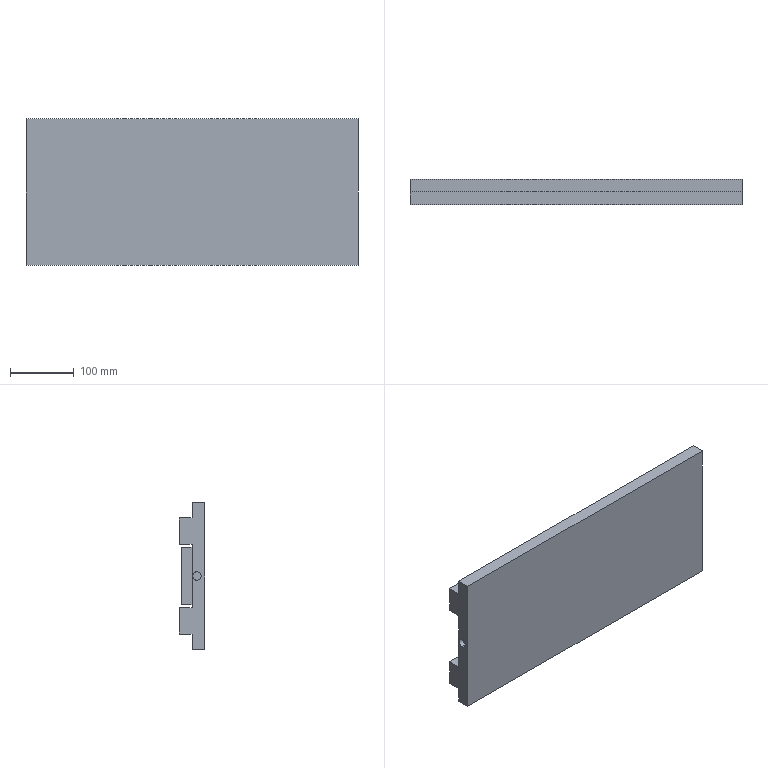Component | SolidWorks | X-AxisSupportBase-1 | 1 solid | 40 faces | box 520 x 40 x 230 mm | volume 3293748 mm3 | plane 27 | cylinder 13 | commonest cylinder face diameters 5.084 x8 13.093 x2 2.946 x2 49.4 x1
STEP:
#1=COLOUR_RGB('',0.7922,0.8196,0.9333);
#2=FILL_AREA_STYLE_COLOUR('',#1);
#3=FILL_AREA_STYLE('',(#2));
#4=SURFACE_STYLE_FILL_AREA(#3);
#5=SURFACE_SIDE_STYLE('',(#4));
#6=SURFACE_STYLE_USAGE(.BOTH.,#5);
#7=PRESENTATION_STYLE_ASSIGNMENT((#6));
#8=CARTESIAN_POINT('',(6.767,1.417,1.368));
#9=VERTEX_POINT('',#8);
#10=CARTESIAN_POINT('',(6.767,1.417,1.568));
#11=VERTEX_POINT('',#10);
#12=CARTESIAN_POINT('',(6.767,1.417,1.468));
#13=DIRECTION('',(0.,1.,0.));
#14=DIRECTION('',(0.,0.,1.));
#15=AXIS2_PLACEMENT_3D('',#12,#13,#14);
#16=CIRCLE('',#15,0.1001);
#17=EDGE_CURVE('',#9,#11,#16,.T.);
#18=ORIENTED_EDGE('',*,*,#17,.T.);
#19=CARTESIAN_POINT('',(6.767,0.7874,1.568));
#20=VERTEX_POINT('',#19);
#21=CARTESIAN_POINT('',(6.767,1.417,1.568));
#22=DIRECTION('',(0.,-1.,0.));
#23=VECTOR('',#22,39.37);
#24=LINE('',#21,#23);
#25=EDGE_CURVE('',#11,#20,#24,.T.);
#26=ORIENTED_EDGE('',*,*,#25,.T.);
#27=CARTESIAN_POINT('',(6.767,0.7874,1.368));
#28=VERTEX_POINT('',#27);
#29=CARTESIAN_POINT('',(6.767,0.7874,1.468));
#30=DIRECTION('',(0.,1.,0.));
#31=DIRECTION('',(0.,0.,1.));
#32=AXIS2_PLACEMENT_3D('',#29,#30,#31);
#33=CIRCLE('',#32,0.1001);
#34=EDGE_CURVE('',#28,#20,#33,.T.);
#35=ORIENTED_EDGE('',*,*,#34,.F.);
#36=CARTESIAN_POINT('',(6.767,1.417,1.368));
#37=DIRECTION('',(0.,-1.,0.));
#38=VECTOR('',#37,39.37);
#39=LINE('',#36,#38);
#40=EDGE_CURVE('',#9,#28,#39,.T.);
#41=ORIENTED_EDGE('',*,*,#40,.F.);
#42=EDGE_LOOP('',(#18,#26,#35,#41));
#43=FACE_OUTER_BOUND('',#42,.T.);
#44=CARTESIAN_POINT('',(6.767,1.417,1.468));
#45=DIRECTION('',(0.,-1.,0.));
#46=DIRECTION('',(0.,0.,-1.));
#47=AXIS2_PLACEMENT_3D('',#44,#45,#46);
#48=CYLINDRICAL_SURFACE('',#47,0.1001);
#49=ADVANCED_FACE('',(#43),#48,.F.);
#50=CARTESIAN_POINT('',(6.208,1.417,1.368));
#51=VERTEX_POINT('',#50);
#52=CARTESIAN_POINT('',(6.208,1.417,1.568));
#53=VERTEX_POINT('',#52);
#54=CARTESIAN_POINT('',(6.208,1.417,1.468));
#55=DIRECTION('',(0.,1.,0.));
#56=DIRECTION('',(0.,0.,1.));
#57=AXIS2_PLACEMENT_3D('',#54,#55,#56);
#58=CIRCLE('',#57,0.1001);
#59=EDGE_CURVE('',#51,#53,#58,.T.);
#60=ORIENTED_EDGE('',*,*,#59,.T.);
#61=CARTESIAN_POINT('',(6.208,0.7874,1.568));
#62=VERTEX_POINT('',#61);
#63=CARTESIAN_POINT('',(6.208,1.417,1.568));
#64=DIRECTION('',(0.,-1.,0.));
#65=VECTOR('',#64,39.37);
#66=LINE('',#63,#65);
#67=EDGE_CURVE('',#53,#62,#66,.T.);
#68=ORIENTED_EDGE('',*,*,#67,.T.);
#69=CARTESIAN_POINT('',(6.208,0.7874,1.368));
#70=VERTEX_POINT('',#69);
#71=CARTESIAN_POINT('',(6.208,0.7874,1.468));
#72=DIRECTION('',(0.,1.,0.));
#73=DIRECTION('',(0.,0.,1.));
#74=AXIS2_PLACEMENT_3D('',#71,#72,#73);
#75=CIRCLE('',#74,0.1001);
#76=EDGE_CURVE('',#70,#62,#75,.T.);
#77=ORIENTED_EDGE('',*,*,#76,.F.);
#78=CARTESIAN_POINT('',(6.208,1.417,1.368));
#79=DIRECTION('',(0.,-1.,0.));
#80=VECTOR('',#79,39.37);
#81=LINE('',#78,#80);
#82=EDGE_CURVE('',#51,#70,#81,.T.);
#83=ORIENTED_EDGE('',*,*,#82,.F.);
#84=EDGE_LOOP('',(#60,#68,#77,#83));
#85=FACE_OUTER_BOUND('',#84,.T.);
#86=CARTESIAN_POINT('',(6.208,1.417,1.468));
#87=DIRECTION('',(0.,-1.,0.));
#88=DIRECTION('',(0.,0.,-1.));
#89=AXIS2_PLACEMENT_3D('',#86,#87,#88);
#90=CYLINDRICAL_SURFACE('',#89,0.1001);
#91=ADVANCED_FACE('',(#85),#90,.F.);
#92=CARTESIAN_POINT('',(6.767,1.417,-1.568));
#93=VERTEX_POINT('',#92);
#94=CARTESIAN_POINT('',(6.767,1.417,-1.368));
#95=VERTEX_POINT('',#94);
#96=CARTESIAN_POINT('',(6.767,1.417,-1.468));
#97=DIRECTION('',(0.,1.,0.));
#98=DIRECTION('',(0.,0.,1.));
#99=AXIS2_PLACEMENT_3D('',#96,#97,#98);
#100=CIRCLE('',#99,0.1001);
#101=EDGE_CURVE('',#93,#95,#100,.T.);
#102=ORIENTED_EDGE('',*,*,#101,.T.);
#103=CARTESIAN_POINT('',(6.767,0.7874,-1.368));
#104=VERTEX_POINT('',#103);
#105=CARTESIAN_POINT('',(6.767,1.417,-1.368));
#106=DIRECTION('',(0.,-1.,0.));
#107=VECTOR('',#106,39.37);
#108=LINE('',#105,#107);
#109=EDGE_CURVE('',#95,#104,#108,.T.);
#110=ORIENTED_EDGE('',*,*,#109,.T.);
#111=CARTESIAN_POINT('',(6.767,0.7874,-1.568));
#112=VERTEX_POINT('',#111);
#113=CARTESIAN_POINT('',(6.767,0.7874,-1.468));
#114=DIRECTION('',(0.,1.,0.));
#115=DIRECTION('',(0.,0.,1.));
#116=AXIS2_PLACEMENT_3D('',#113,#114,#115);
#117=CIRCLE('',#116,0.1001);
#118=EDGE_CURVE('',#112,#104,#117,.T.);
#119=ORIENTED_EDGE('',*,*,#118,.F.);
#120=CARTESIAN_POINT('',(6.767,1.417,-1.568));
#121=DIRECTION('',(0.,-1.,0.));
#122=VECTOR('',#121,39.37);
#123=LINE('',#120,#122);
#124=EDGE_CURVE('',#93,#112,#123,.T.);
#125=ORIENTED_EDGE('',*,*,#124,.F.);
#126=EDGE_LOOP('',(#102,#110,#119,#125));
#127=FACE_OUTER_BOUND('',#126,.T.);
#128=CARTESIAN_POINT('',(6.767,1.417,-1.468));
#129=DIRECTION('',(0.,-1.,0.));
#130=DIRECTION('',(0.,0.,-1.));
#131=AXIS2_PLACEMENT_3D('',#128,#129,#130);
#132=CYLINDRICAL_SURFACE('',#131,0.1001);
#133=ADVANCED_FACE('',(#127),#132,.F.);
#134=CARTESIAN_POINT('',(6.208,1.417,-1.568));
#135=VERTEX_POINT('',#134);
#136=CARTESIAN_POINT('',(6.208,1.417,-1.368));
#137=VERTEX_POINT('',#136);
#138=CARTESIAN_POINT('',(6.208,1.417,-1.468));
#139=DIRECTION('',(0.,1.,0.));
#140=DIRECTION('',(0.,0.,1.));
#141=AXIS2_PLACEMENT_3D('',#138,#139,#140);
#142=CIRCLE('',#141,0.1001);
#143=EDGE_CURVE('',#135,#137,#142,.T.);
#144=ORIENTED_EDGE('',*,*,#143,.T.);
#145=CARTESIAN_POINT('',(6.208,0.7874,-1.368));
#146=VERTEX_POINT('',#145);
#147=CARTESIAN_POINT('',(6.208,1.417,-1.368));
#148=DIRECTION('',(0.,-1.,0.));
#149=VECTOR('',#148,39.37);
#150=LINE('',#147,#149);
#151=EDGE_CURVE('',#137,#146,#150,.T.);
#152=ORIENTED_EDGE('',*,*,#151,.T.);
#153=CARTESIAN_POINT('',(6.208,0.7874,-1.568));
#154=VERTEX_POINT('',#153);
#155=CARTESIAN_POINT('',(6.208,0.7874,-1.468));
#156=DIRECTION('',(0.,1.,0.));
#157=DIRECTION('',(0.,0.,1.));
#158=AXIS2_PLACEMENT_3D('',#155,#156,#157);
#159=CIRCLE('',#158,0.1001);
#160=EDGE_CURVE('',#154,#146,#159,.T.);
#161=ORIENTED_EDGE('',*,*,#160,.F.);
#162=CARTESIAN_POINT('',(6.208,1.417,-1.568));
#163=DIRECTION('',(0.,-1.,0.));
#164=VECTOR('',#163,39.37);
#165=LINE('',#162,#164);
#166=EDGE_CURVE('',#135,#154,#165,.T.);
#167=ORIENTED_EDGE('',*,*,#166,.F.);
#168=EDGE_LOOP('',(#144,#152,#161,#167));
#169=FACE_OUTER_BOUND('',#168,.T.);
#170=CARTESIAN_POINT('',(6.208,1.417,-1.468));
#171=DIRECTION('',(0.,-1.,0.));
#172=DIRECTION('',(0.,0.,-1.));
#173=AXIS2_PLACEMENT_3D('',#170,#171,#172);
#174=CYLINDRICAL_SURFACE('',#173,0.1001);
#175=ADVANCED_FACE('',(#169),#174,.F.);
#176=CARTESIAN_POINT('',(-10.591,0.4812,-0.2577));
#177=VERTEX_POINT('',#176);
#178=CARTESIAN_POINT('',(-10.591,0.4812,0.2577));
#179=VERTEX_POINT('',#178);
#180=CARTESIAN_POINT('',(-10.591,0.4812,0.));
#181=DIRECTION('',(-1.,0.,0.));
#182=DIRECTION('',(0.,0.,1.));
#183=AXIS2_PLACEMENT_3D('',#180,#181,#182);
#184=CIRCLE('',#183,0.2577);
#185=EDGE_CURVE('',#177,#179,#184,.T.);
#186=ORIENTED_EDGE('',*,*,#185,.F.);
#187=CARTESIAN_POINT('',(-10.906,0.4812,-0.2577));
#188=VERTEX_POINT('',#187);
#189=CARTESIAN_POINT('',(-10.591,0.4812,-0.2577));
#190=DIRECTION('',(-1.,0.,0.));
#191=VECTOR('',#190,39.37);
#192=LINE('',#189,#191);
#193=EDGE_CURVE('',#177,#188,#192,.T.);
#194=ORIENTED_EDGE('',*,*,#193,.T.);
#195=CARTESIAN_POINT('',(-10.906,0.4812,0.2577));
#196=VERTEX_POINT('',#195);
#197=CARTESIAN_POINT('',(-10.906,0.4812,0.));
#198=DIRECTION('',(-1.,0.,0.));
#199=DIRECTION('',(0.,0.,1.));
#200=AXIS2_PLACEMENT_3D('',#197,#198,#199);
#201=CIRCLE('',#200,0.2577);
#202=EDGE_CURVE('',#188,#196,#201,.T.);
#203=ORIENTED_EDGE('',*,*,#202,.T.);
#204=CARTESIAN_POINT('',(-10.591,0.4812,0.2577));
#205=DIRECTION('',(-1.,0.,0.));
#206=VECTOR('',#205,39.37);
#207=LINE('',#204,#206);
#208=EDGE_CURVE('',#179,#196,#207,.T.);
#209=ORIENTED_EDGE('',*,*,#208,.F.);
#210=EDGE_LOOP('',(#186,#194,#203,#209));
#211=FACE_OUTER_BOUND('',#210,.T.);
#212=CARTESIAN_POINT('',(-10.591,0.4812,0.));
#213=DIRECTION('',(-1.,0.,0.));
#214=DIRECTION('',(0.,0.,1.));
#215=AXIS2_PLACEMENT_3D('',#212,#213,#214);
#216=CYLINDRICAL_SURFACE('',#215,0.2577);
#217=ADVANCED_FACE('',(#211),#216,.F.);
#218=CARTESIAN_POINT('',(7.039,1.417,0.191));
#219=VERTEX_POINT('',#218);
#220=CARTESIAN_POINT('',(7.039,1.417,-0.191));
#221=VERTEX_POINT('',#220);
#222=CARTESIAN_POINT('',(7.039,2.371,0.));
#223=DIRECTION('',(1.,0.,0.));
#224=DIRECTION('',(0.,0.,-1.));
#225=AXIS2_PLACEMENT_3D('',#222,#223,#224);
#226=CIRCLE('',#225,0.9724);
#227=EDGE_CURVE('',#219,#221,#226,.T.);
#228=ORIENTED_EDGE('',*,*,#227,.F.);
#229=CARTESIAN_POINT('',(7.039,1.417,1.781));
#230=VERTEX_POINT('',#229);
#231=CARTESIAN_POINT('',(7.039,1.417,-1.083));
#232=DIRECTION('',(0.,0.,-1.));
#233=VECTOR('',#232,39.37);
#234=LINE('',#231,#233);
#235=EDGE_CURVE('',#230,#219,#234,.T.);
#236=ORIENTED_EDGE('',*,*,#235,.F.);
#237=CARTESIAN_POINT('',(7.039,0.7874,1.781));
#238=VERTEX_POINT('',#237);
#239=CARTESIAN_POINT('',(7.039,1.417,1.781));
#240=DIRECTION('',(0.,-1.,0.));
#241=VECTOR('',#240,39.37);
#242=LINE('',#239,#241);
#243=EDGE_CURVE('',#230,#238,#242,.T.);
#244=ORIENTED_EDGE('',*,*,#243,.T.);
#245=CARTESIAN_POINT('',(7.039,0.7874,-1.781));
#246=VERTEX_POINT('',#245);
#247=CARTESIAN_POINT('',(7.039,0.7874,1.791));
#248=DIRECTION('',(0.,0.,-1.));
#249=VECTOR('',#248,39.37);
#250=LINE('',#247,#249);
#251=EDGE_CURVE('',#238,#246,#250,.T.);
#252=ORIENTED_EDGE('',*,*,#251,.T.);
#253=CARTESIAN_POINT('',(7.039,1.417,-1.781));
#254=VERTEX_POINT('',#253);
#255=CARTESIAN_POINT('',(7.039,1.417,-1.781));
#256=DIRECTION('',(0.,1.,0.));
#257=VECTOR('',#256,39.37);
#258=LINE('',#255,#257);
#259=EDGE_CURVE('',#246,#254,#258,.T.);
#260=ORIENTED_EDGE('',*,*,#259,.T.);
#261=CARTESIAN_POINT('',(7.039,1.417,-1.083));
#262=DIRECTION('',(0.,0.,-1.));
#263=VECTOR('',#262,39.37);
#264=LINE('',#261,#263);
#265=EDGE_CURVE('',#221,#254,#264,.T.);
#266=ORIENTED_EDGE('',*,*,#265,.F.);
#267=EDGE_LOOP('',(#228,#236,#244,#252,#260,#266));
#268=FACE_OUTER_BOUND('',#267,.T.);
#269=CARTESIAN_POINT('',(7.039,1.417,1.791));
#270=DIRECTION('',(-1.,0.,0.));
#271=DIRECTION('',(0.,0.,1.));
#272=AXIS2_PLACEMENT_3D('',#269,#270,#271);
#273=PLANE('',#272);
#274=ADVANCED_FACE('',(#268),#273,.F.);
#275=CARTESIAN_POINT('',(-10.906,0.7874,4.528));
#276=VERTEX_POINT('',#275);
#277=CARTESIAN_POINT('',(9.567,0.7874,4.528));
#278=VERTEX_POINT('',#277);
#279=CARTESIAN_POINT('',(0.,0.7874,4.528));
#280=DIRECTION('',(1.,0.,0.));
#281=VECTOR('',#280,39.37);
#282=LINE('',#279,#281);
#283=EDGE_CURVE('',#276,#278,#282,.T.);
#284=ORIENTED_EDGE('',*,*,#283,.T.);
#285=CARTESIAN_POINT('',(9.567,0.7874,3.579));
#286=VERTEX_POINT('',#285);
#287=CARTESIAN_POINT('',(9.567,0.7874,0.));
#288=DIRECTION('',(0.,0.,1.));
#289=VECTOR('',#288,39.37);
#290=LINE('',#287,#289);
#291=EDGE_CURVE('',#286,#278,#290,.T.);
#292=ORIENTED_EDGE('',*,*,#291,.F.);
#293=CARTESIAN_POINT('',(-10.906,0.7874,3.579));
#294=VERTEX_POINT('',#293);
#295=CARTESIAN_POINT('',(0.,0.7874,3.579));
#296=DIRECTION('',(1.,0.,0.));
#297=VECTOR('',#296,39.37);
#298=LINE('',#295,#297);
#299=EDGE_CURVE('',#294,#286,#298,.T.);
#300=ORIENTED_EDGE('',*,*,#299,.F.);
#301=CARTESIAN_POINT('',(-10.906,0.7874,4.528));
#302=DIRECTION('',(0.,0.,1.));
#303=VECTOR('',#302,39.37);
#304=LINE('',#301,#303);
#305=EDGE_CURVE('',#294,#276,#304,.T.);
#306=ORIENTED_EDGE('',*,*,#305,.T.);
#307=EDGE_LOOP('',(#284,#292,#300,#306));
#308=FACE_OUTER_BOUND('',#307,.T.);
#309=CARTESIAN_POINT('',(0.,0.7874,0.));
#310=DIRECTION('',(0.,-1.,0.));
#311=DIRECTION('',(0.,0.,-1.));
#312=AXIS2_PLACEMENT_3D('',#309,#310,#311);
#313=PLANE('',#312);
#314=ADVANCED_FACE('',(#308),#313,.F.);
#315=CARTESIAN_POINT('',(9.567,0.7874,-4.528));
#316=VERTEX_POINT('',#315);
#317=CARTESIAN_POINT('',(-10.906,0.7874,-4.528));
#318=VERTEX_POINT('',#317);
#319=CARTESIAN_POINT('',(-0.,0.7874,-4.528));
#320=DIRECTION('',(-1.,0.,0.));
#321=VECTOR('',#320,39.37);
#322=LINE('',#319,#321);
#323=EDGE_CURVE('',#316,#318,#322,.T.);
#324=ORIENTED_EDGE('',*,*,#323,.T.);
#325=CARTESIAN_POINT('',(-10.906,0.7874,-3.579));
#326=VERTEX_POINT('',#325);
#327=CARTESIAN_POINT('',(-10.906,0.7874,4.528));
#328=DIRECTION('',(0.,0.,1.));
#329=VECTOR('',#328,39.37);
#330=LINE('',#327,#329);
#331=EDGE_CURVE('',#318,#326,#330,.T.);
#332=ORIENTED_EDGE('',*,*,#331,.T.);
#333=CARTESIAN_POINT('',(9.567,0.7874,-3.579));
#334=VERTEX_POINT('',#333);
#335=CARTESIAN_POINT('',(0.,0.7874,-3.579));
#336=DIRECTION('',(1.,0.,0.));
#337=VECTOR('',#336,39.37);
#338=LINE('',#335,#337);
#339=EDGE_CURVE('',#326,#334,#338,.T.);
#340=ORIENTED_EDGE('',*,*,#339,.T.);
#341=CARTESIAN_POINT('',(9.567,0.7874,0.));
#342=DIRECTION('',(0.,0.,1.));
#343=VECTOR('',#342,39.37);
#344=LINE('',#341,#343);
#345=EDGE_CURVE('',#316,#334,#344,.T.);
#346=ORIENTED_EDGE('',*,*,#345,.F.);
#347=EDGE_LOOP('',(#324,#332,#340,#346));
#348=FACE_OUTER_BOUND('',#347,.T.);
#349=CARTESIAN_POINT('',(0.,0.7874,0.));
#350=DIRECTION('',(0.,-1.,0.));
#351=DIRECTION('',(0.,0.,-1.));
#352=AXIS2_PLACEMENT_3D('',#349,#350,#351);
#353=PLANE('',#352);
#354=ADVANCED_FACE('',(#348),#353,.F.);
#355=CARTESIAN_POINT('',(9.567,0.,4.528));
#356=VERTEX_POINT('',#355);
#357=CARTESIAN_POINT('',(9.567,0.,-4.528));
#358=VERTEX_POINT('',#357);
#359=CARTESIAN_POINT('',(9.567,0.,0.));
#360=DIRECTION('',(0.,0.,-1.));
#361=VECTOR('',#360,39.37);
#362=LINE('',#359,#361);
#363=EDGE_CURVE('',#356,#358,#362,.T.);
#364=ORIENTED_EDGE('',*,*,#363,.F.);
#365=CARTESIAN_POINT('',(-10.906,0.,4.528));
#366=VERTEX_POINT('',#365);
#367=CARTESIAN_POINT('',(0.,0.,4.528));
#368=DIRECTION('',(-1.,0.,0.));
#369=VECTOR('',#368,39.37);
#370=LINE('',#367,#369);
#371=EDGE_CURVE('',#356,#366,#370,.T.);
#372=ORIENTED_EDGE('',*,*,#371,.T.);
#373=CARTESIAN_POINT('',(-10.906,0.,-4.528));
#374=VERTEX_POINT('',#373);
#375=CARTESIAN_POINT('',(-10.906,0.,4.528));
#376=DIRECTION('',(0.,0.,1.));
#377=VECTOR('',#376,39.37);
#378=LINE('',#375,#377);
#379=EDGE_CURVE('',#374,#366,#378,.T.);
#380=ORIENTED_EDGE('',*,*,#379,.F.);
#381=CARTESIAN_POINT('',(-0.,0.,-4.528));
#382=DIRECTION('',(1.,0.,-0.));
#383=VECTOR('',#382,39.37);
#384=LINE('',#381,#383);
#385=EDGE_CURVE('',#374,#358,#384,.T.);
#386=ORIENTED_EDGE('',*,*,#385,.T.);
#387=EDGE_LOOP('',(#364,#372,#380,#386));
#388=FACE_OUTER_BOUND('',#387,.T.);
#389=CARTESIAN_POINT('',(0.,0.,0.));
#390=DIRECTION('',(0.,-1.,0.));
#391=DIRECTION('',(0.,0.,-1.));
#392=AXIS2_PLACEMENT_3D('',#389,#390,#391);
#393=PLANE('',#392);
#394=ADVANCED_FACE('',(#388),#393,.T.);
#395=CARTESIAN_POINT('',(-10.906,0.4812,0.));
#396=DIRECTION('',(-1.,0.,0.));
#397=DIRECTION('',(0.,0.,1.));
#398=AXIS2_PLACEMENT_3D('',#395,#396,#397);
#399=CIRCLE('',#398,0.2577);
#400=EDGE_CURVE('',#196,#188,#399,.T.);
#401=ORIENTED_EDGE('',*,*,#400,.F.);
#402=ORIENTED_EDGE('',*,*,#202,.F.);
#403=EDGE_LOOP('',(#401,#402));
#404=FACE_BOUND('',#403,.T.);
#405=CARTESIAN_POINT('',(-10.906,-11.22,4.528));
#406=DIRECTION('',(0.,1.,0.));
#407=VECTOR('',#406,39.37);
#408=LINE('',#405,#407);
#409=EDGE_CURVE('',#366,#276,#408,.T.);
#410=ORIENTED_EDGE('',*,*,#409,.T.);
#411=ORIENTED_EDGE('',*,*,#305,.F.);
#412=CARTESIAN_POINT('',(-10.906,1.575,3.579));
#413=VERTEX_POINT('',#412);
#414=CARTESIAN_POINT('',(-10.906,1.575,3.579));
#415=DIRECTION('',(0.,-1.,0.));
#416=VECTOR('',#415,39.37);
#417=LINE('',#414,#416);
#418=EDGE_CURVE('',#413,#294,#417,.T.);
#419=ORIENTED_EDGE('',*,*,#418,.F.);
#420=CARTESIAN_POINT('',(-10.906,1.575,1.945));
#421=VERTEX_POINT('',#420);
#422=CARTESIAN_POINT('',(-10.906,1.575,0.));
#423=DIRECTION('',(0.,0.,1.));
#424=VECTOR('',#423,39.37);
#425=LINE('',#422,#424);
#426=EDGE_CURVE('',#421,#413,#425,.T.);
#427=ORIENTED_EDGE('',*,*,#426,.F.);
#428=CARTESIAN_POINT('',(-10.906,0.8454,1.945));
#429=VERTEX_POINT('',#428);
#430=CARTESIAN_POINT('',(-10.906,0.,1.945));
#431=DIRECTION('',(0.,-1.,0.));
#432=VECTOR('',#431,39.37);
#433=LINE('',#430,#432);
#434=EDGE_CURVE('',#421,#429,#433,.T.);
#435=ORIENTED_EDGE('',*,*,#434,.T.);
#436=CARTESIAN_POINT('',(-10.906,0.7952,1.916));
#437=VERTEX_POINT('',#436);
#438=CARTESIAN_POINT('',(-10.906,0.8454,1.887));
#439=DIRECTION('',(1.,0.,0.));
#440=DIRECTION('',(0.,0.,-1.));
#441=AXIS2_PLACEMENT_3D('',#438,#439,#440);
#442=CIRCLE('',#441,0.058);
#443=EDGE_CURVE('',#429,#437,#442,.T.);
#444=ORIENTED_EDGE('',*,*,#443,.T.);
#445=CARTESIAN_POINT('',(-10.906,0.7874,1.916));
#446=VERTEX_POINT('',#445);
#447=CARTESIAN_POINT('',(-10.906,1.575,1.916));
#448=DIRECTION('',(0.,-1.,0.));
#449=VECTOR('',#448,39.37);
#450=LINE('',#447,#449);
#451=EDGE_CURVE('',#437,#446,#450,.T.);
#452=ORIENTED_EDGE('',*,*,#451,.T.);
#453=CARTESIAN_POINT('',(-10.906,0.7874,-1.916));
#454=VERTEX_POINT('',#453);
#455=CARTESIAN_POINT('',(-10.906,0.7874,4.528));
#456=DIRECTION('',(0.,0.,1.));
#457=VECTOR('',#456,39.37);
#458=LINE('',#455,#457);
#459=EDGE_CURVE('',#454,#446,#458,.T.);
#460=ORIENTED_EDGE('',*,*,#459,.F.);
#461=CARTESIAN_POINT('',(-10.906,0.7952,-1.916));
#462=VERTEX_POINT('',#461);
#463=CARTESIAN_POINT('',(-10.906,1.575,-1.916));
#464=DIRECTION('',(0.,-1.,0.));
#465=VECTOR('',#464,39.37);
#466=LINE('',#463,#465);
#467=EDGE_CURVE('',#462,#454,#466,.T.);
#468=ORIENTED_EDGE('',*,*,#467,.F.);
#469=CARTESIAN_POINT('',(-10.906,0.8454,-1.945));
#470=VERTEX_POINT('',#469);
#471=CARTESIAN_POINT('',(-10.906,0.8454,-1.887));
#472=DIRECTION('',(-1.,0.,0.));
#473=DIRECTION('',(0.,0.,1.));
#474=AXIS2_PLACEMENT_3D('',#471,#472,#473);
#475=CIRCLE('',#474,0.058);
#476=EDGE_CURVE('',#470,#462,#475,.T.);
#477=ORIENTED_EDGE('',*,*,#476,.F.);
#478=CARTESIAN_POINT('',(-10.906,1.575,-1.945));
#479=VERTEX_POINT('',#478);
#480=CARTESIAN_POINT('',(-10.906,0.,-1.945));
#481=DIRECTION('',(0.,-1.,-0.));
#482=VECTOR('',#481,39.37);
#483=LINE('',#480,#482);
#484=EDGE_CURVE('',#479,#470,#483,.T.);
#485=ORIENTED_EDGE('',*,*,#484,.F.);
#486=CARTESIAN_POINT('',(-10.906,1.575,-3.579));
#487=VERTEX_POINT('',#486);
#488=CARTESIAN_POINT('',(-10.906,1.575,0.));
#489=DIRECTION('',(0.,0.,1.));
#490=VECTOR('',#489,39.37);
#491=LINE('',#488,#490);
#492=EDGE_CURVE('',#487,#479,#491,.T.);
#493=ORIENTED_EDGE('',*,*,#492,.F.);
#494=CARTESIAN_POINT('',(-10.906,1.575,-3.579));
#495=DIRECTION('',(0.,-1.,0.));
#496=VECTOR('',#495,39.37);
#497=LINE('',#494,#496);
#498=EDGE_CURVE('',#487,#326,#497,.T.);
#499=ORIENTED_EDGE('',*,*,#498,.T.);
#500=ORIENTED_EDGE('',*,*,#331,.F.);
#501=CARTESIAN_POINT('',(-10.906,-11.22,-4.528));
#502=DIRECTION('',(0.,1.,0.));
#503=VECTOR('',#502,39.37);
#504=LINE('',#501,#503);
#505=EDGE_CURVE('',#374,#318,#504,.T.);
#506=ORIENTED_EDGE('',*,*,#505,.F.);
#507=ORIENTED_EDGE('',*,*,#379,.T.);
#508=EDGE_LOOP('',(#410,#411,#419,#427,#435,#444,#452,#460,#468,#477,#485,#493,#499,#500,#506,#507));
#509=FACE_OUTER_BOUND('',#508,.T.);
#510=CARTESIAN_POINT('',(-10.906,0.7874,4.528));
#511=DIRECTION('',(1.,0.,0.));
#512=DIRECTION('',(0.,0.,-1.));
#513=AXIS2_PLACEMENT_3D('',#510,#511,#512);
#514=PLANE('',#513);
#515=ADVANCED_FACE('',(#404,#509),#514,.F.);
#516=ORIENTED_EDGE('',*,*,#291,.T.);
#517=CARTESIAN_POINT('',(9.567,0.,4.528));
#518=DIRECTION('',(0.,-1.,0.));
#519=VECTOR('',#518,39.37);
#520=LINE('',#517,#519);
#521=EDGE_CURVE('',#278,#356,#520,.T.);
#522=ORIENTED_EDGE('',*,*,#521,.T.);
#523=ORIENTED_EDGE('',*,*,#363,.T.);
#524=CARTESIAN_POINT('',(9.567,0.,-4.528));
#525=DIRECTION('',(0.,1.,0.));
#526=VECTOR('',#525,39.37);
#527=LINE('',#524,#526);
#528=EDGE_CURVE('',#358,#316,#527,.T.);
#529=ORIENTED_EDGE('',*,*,#528,.T.);
#530=ORIENTED_EDGE('',*,*,#345,.T.);
#531=CARTESIAN_POINT('',(9.567,1.575,-3.579));
#532=VERTEX_POINT('',#531);
#533=CARTESIAN_POINT('',(9.567,1.575,-3.579));
#534=DIRECTION('',(0.,-1.,0.));
#535=VECTOR('',#534,39.37);
#536=LINE('',#533,#535);
#537=EDGE_CURVE('',#532,#334,#536,.T.);
#538=ORIENTED_EDGE('',*,*,#537,.F.);
#539=CARTESIAN_POINT('',(9.567,1.575,-1.945));
#540=VERTEX_POINT('',#539);
#541=CARTESIAN_POINT('',(9.567,1.575,0.));
#542=DIRECTION('',(0.,0.,-1.));
#543=VECTOR('',#542,39.37);
#544=LINE('',#541,#543);
#545=EDGE_CURVE('',#540,#532,#544,.T.);
#546=ORIENTED_EDGE('',*,*,#545,.F.);
#547=CARTESIAN_POINT('',(9.567,0.8454,-1.945));
#548=VERTEX_POINT('',#547);
#549=CARTESIAN_POINT('',(9.567,0.,-1.945));
#550=DIRECTION('',(0.,-1.,-0.));
#551=VECTOR('',#550,39.37);
#552=LINE('',#549,#551);
#553=EDGE_CURVE('',#540,#548,#552,.T.);
#554=ORIENTED_EDGE('',*,*,#553,.T.);
#555=CARTESIAN_POINT('',(9.567,0.7952,-1.916));
#556=VERTEX_POINT('',#555);
#557=CARTESIAN_POINT('',(9.567,0.8454,-1.887));
#558=DIRECTION('',(-1.,0.,0.));
#559=DIRECTION('',(0.,0.,-1.));
#560=AXIS2_PLACEMENT_3D('',#557,#558,#559);
#561=CIRCLE('',#560,0.058);
#562=EDGE_CURVE('',#548,#556,#561,.T.);
#563=ORIENTED_EDGE('',*,*,#562,.T.);
#564=CARTESIAN_POINT('',(9.567,0.7874,-1.916));
#565=VERTEX_POINT('',#564);
#566=CARTESIAN_POINT('',(9.567,-3.383,-1.916));
#567=DIRECTION('',(0.,1.,0.));
#568=VECTOR('',#567,39.37);
#569=LINE('',#566,#568);
#570=EDGE_CURVE('',#565,#556,#569,.T.);
#571=ORIENTED_EDGE('',*,*,#570,.F.);
#572=CARTESIAN_POINT('',(9.567,0.7874,1.916));
#573=VERTEX_POINT('',#572);
#574=CARTESIAN_POINT('',(9.567,0.7874,1.916));
#575=DIRECTION('',(-0.,0.,-1.));
#576=VECTOR('',#575,39.37);
#577=LINE('',#574,#576);
#578=EDGE_CURVE('',#573,#565,#577,.T.);
#579=ORIENTED_EDGE('',*,*,#578,.F.);
#580=CARTESIAN_POINT('',(9.567,0.7952,1.916));
#581=VERTEX_POINT('',#580);
#582=CARTESIAN_POINT('',(9.567,-3.383,1.916));
#583=DIRECTION('',(0.,1.,0.));
#584=VECTOR('',#583,39.37);
#585=LINE('',#582,#584);
#586=EDGE_CURVE('',#573,#581,#585,.T.);
#587=ORIENTED_EDGE('',*,*,#586,.T.);
#588=CARTESIAN_POINT('',(9.567,0.8454,1.945));
#589=VERTEX_POINT('',#588);
#590=CARTESIAN_POINT('',(9.567,0.8454,1.887));
#591=DIRECTION('',(1.,0.,0.));
#592=DIRECTION('',(0.,0.,-1.));
#593=AXIS2_PLACEMENT_3D('',#590,#591,#592);
#594=CIRCLE('',#593,0.058);
#595=EDGE_CURVE('',#589,#581,#594,.T.);
#596=ORIENTED_EDGE('',*,*,#595,.F.);
#597=CARTESIAN_POINT('',(9.567,1.575,1.945));
#598=VERTEX_POINT('',#597);
#599=CARTESIAN_POINT('',(9.567,0.,1.945));
#600=DIRECTION('',(0.,-1.,0.));
#601=VECTOR('',#600,39.37);
#602=LINE('',#599,#601);
#603=EDGE_CURVE('',#598,#589,#602,.T.);
#604=ORIENTED_EDGE('',*,*,#603,.F.);
#605=CARTESIAN_POINT('',(9.567,1.575,3.579));
#606=VERTEX_POINT('',#605);
#607=CARTESIAN_POINT('',(9.567,1.575,0.));
#608=DIRECTION('',(0.,0.,-1.));
#609=VECTOR('',#608,39.37);
#610=LINE('',#607,#609);
#611=EDGE_CURVE('',#606,#598,#610,.T.);
#612=ORIENTED_EDGE('',*,*,#611,.F.);
#613=CARTESIAN_POINT('',(9.567,1.575,3.579));
#614=DIRECTION('',(0.,-1.,0.));
#615=VECTOR('',#614,39.37);
#616=LINE('',#613,#615);
#617=EDGE_CURVE('',#606,#286,#616,.T.);
#618=ORIENTED_EDGE('',*,*,#617,.T.);
#619=EDGE_LOOP('',(#516,#522,#523,#529,#530,#538,#546,#554,#563,#571,#579,#587,#596,#604,#612,#618));
#620=FACE_OUTER_BOUND('',#619,.T.);
#621=CARTESIAN_POINT('',(9.567,0.,0.));
#622=DIRECTION('',(1.,0.,0.));
#623=DIRECTION('',(0.,0.,-1.));
#624=AXIS2_PLACEMENT_3D('',#621,#622,#623);
#625=PLANE('',#624);
#626=ADVANCED_FACE('',(#620),#625,.T.);
#627=CARTESIAN_POINT('',(0.,1.575,3.579));
#628=DIRECTION('',(1.,0.,0.));
#629=VECTOR('',#628,39.37);
#630=LINE('',#627,#629);
#631=EDGE_CURVE('',#413,#606,#630,.T.);
#632=ORIENTED_EDGE('',*,*,#631,.T.);
#633=ORIENTED_EDGE('',*,*,#611,.T.);
#634=CARTESIAN_POINT('',(0.,1.575,1.945));
#635=DIRECTION('',(-1.,0.,0.));
#636=VECTOR('',#635,39.37);
#637=LINE('',#634,#636);
#638=EDGE_CURVE('',#598,#421,#637,.T.);
#639=ORIENTED_EDGE('',*,*,#638,.T.);
#640=ORIENTED_EDGE('',*,*,#426,.T.);
#641=EDGE_LOOP('',(#632,#633,#639,#640));
#642=FACE_OUTER_BOUND('',#641,.T.);
#643=CARTESIAN_POINT('',(0.,1.575,0.));
#644=DIRECTION('',(0.,1.,0.));
#645=DIRECTION('',(0.,0.,1.));
#646=AXIS2_PLACEMENT_3D('',#643,#644,#645);
#647=PLANE('',#646);
#648=ADVANCED_FACE('',(#642),#647,.T.);
#649=CARTESIAN_POINT('',(0.,1.575,-3.579));
#650=DIRECTION('',(1.,0.,0.));
#651=VECTOR('',#650,39.37);
#652=LINE('',#649,#651);
#653=EDGE_CURVE('',#487,#532,#652,.T.);
#654=ORIENTED_EDGE('',*,*,#653,.T.);
#655=ORIENTED_EDGE('',*,*,#537,.T.);
#656=ORIENTED_EDGE('',*,*,#339,.F.);
#657=ORIENTED_EDGE('',*,*,#498,.F.);
#658=EDGE_LOOP('',(#654,#655,#656,#657));
#659=FACE_OUTER_BOUND('',#658,.T.);
#660=CARTESIAN_POINT('',(0.,1.575,-3.579));
#661=DIRECTION('',(0.,0.,-1.));
#662=DIRECTION('',(-1.,0.,0.));
#663=AXIS2_PLACEMENT_3D('',#660,#661,#662);
#664=PLANE('',#663);
#665=ADVANCED_FACE('',(#659),#664,.T.);
#666=CARTESIAN_POINT('',(0.,1.575,-1.945));
#667=DIRECTION('',(-1.,0.,0.));
#668=VECTOR('',#667,39.37);
#669=LINE('',#666,#668);
#670=EDGE_CURVE('',#540,#479,#669,.T.);
#671=ORIENTED_EDGE('',*,*,#670,.F.);
#672=ORIENTED_EDGE('',*,*,#545,.T.);
#673=ORIENTED_EDGE('',*,*,#653,.F.);
#674=ORIENTED_EDGE('',*,*,#492,.T.);
#675=EDGE_LOOP('',(#671,#672,#673,#674));
#676=FACE_OUTER_BOUND('',#675,.T.);
#677=CARTESIAN_POINT('',(0.,1.575,0.));
#678=DIRECTION('',(0.,1.,0.));
#679=DIRECTION('',(0.,0.,1.));
#680=AXIS2_PLACEMENT_3D('',#677,#678,#679);
#681=PLANE('',#680);
#682=ADVANCED_FACE('',(#676),#681,.T.);
#683=ORIENTED_EDGE('',*,*,#617,.F.);
#684=ORIENTED_EDGE('',*,*,#631,.F.);
#685=ORIENTED_EDGE('',*,*,#418,.T.);
#686=ORIENTED_EDGE('',*,*,#299,.T.);
#687=EDGE_LOOP('',(#683,#684,#685,#686));
#688=FACE_OUTER_BOUND('',#687,.T.);
#689=CARTESIAN_POINT('',(0.,1.575,3.579));
#690=DIRECTION('',(0.,0.,-1.));
#691=DIRECTION('',(-1.,0.,0.));
#692=AXIS2_PLACEMENT_3D('',#689,#690,#691);
#693=PLANE('',#692);
#694=ADVANCED_FACE('',(#688),#693,.F.);
#695=ORIENTED_EDGE('',*,*,#562,.F.);
#696=CARTESIAN_POINT('',(19.803,0.8454,-1.945));
#697=DIRECTION('',(-1.,0.,0.));
#698=VECTOR('',#697,39.37);
#699=LINE('',#696,#698);
#700=EDGE_CURVE('',#548,#470,#699,.T.);
#701=ORIENTED_EDGE('',*,*,#700,.T.);
#702=ORIENTED_EDGE('',*,*,#476,.T.);
#703=CARTESIAN_POINT('',(19.803,0.7952,-1.916));
#704=DIRECTION('',(-1.,0.,0.));
#705=VECTOR('',#704,39.37);
#706=LINE('',#703,#705);
#707=EDGE_CURVE('',#556,#462,#706,.T.);
#708=ORIENTED_EDGE('',*,*,#707,.F.);
#709=EDGE_LOOP('',(#695,#701,#702,#708));
#710=FACE_OUTER_BOUND('',#709,.T.);
#711=CARTESIAN_POINT('',(19.803,0.8454,-1.887));
#712=DIRECTION('',(-1.,0.,0.));
#713=DIRECTION('',(0.,0.,1.));
#714=AXIS2_PLACEMENT_3D('',#711,#712,#713);
#715=CYLINDRICAL_SURFACE('',#714,0.058);
#716=ADVANCED_FACE('',(#710),#715,.F.);
#717=ORIENTED_EDGE('',*,*,#553,.F.);
#718=ORIENTED_EDGE('',*,*,#670,.T.);
#719=ORIENTED_EDGE('',*,*,#484,.T.);
#720=ORIENTED_EDGE('',*,*,#700,.F.);
#721=EDGE_LOOP('',(#717,#718,#719,#720));
#722=FACE_OUTER_BOUND('',#721,.T.);
#723=CARTESIAN_POINT('',(19.803,0.,-1.945));
#724=DIRECTION('',(0.,0.,-1.));
#725=DIRECTION('',(0.,1.,0.));
#726=AXIS2_PLACEMENT_3D('',#723,#724,#725);
#727=PLANE('',#726);
#728=ADVANCED_FACE('',(#722),#727,.F.);
#729=CARTESIAN_POINT('',(19.803,0.8454,1.945));
#730=DIRECTION('',(-1.,0.,0.));
#731=VECTOR('',#730,39.37);
#732=LINE('',#729,#731);
#733=EDGE_CURVE('',#589,#429,#732,.T.);
#734=ORIENTED_EDGE('',*,*,#733,.F.);
#735=ORIENTED_EDGE('',*,*,#595,.T.);
#736=CARTESIAN_POINT('',(19.803,0.7952,1.916));
#737=DIRECTION('',(-1.,0.,0.));
#738=VECTOR('',#737,39.37);
#739=LINE('',#736,#738);
#740=EDGE_CURVE('',#581,#437,#739,.T.);
#741=ORIENTED_EDGE('',*,*,#740,.T.);
#742=ORIENTED_EDGE('',*,*,#443,.F.);
#743=EDGE_LOOP('',(#734,#735,#741,#742));
#744=FACE_OUTER_BOUND('',#743,.T.);
#745=CARTESIAN_POINT('',(19.803,0.8454,1.887));
#746=DIRECTION('',(-1.,0.,0.));
#747=DIRECTION('',(0.,0.,1.));
#748=AXIS2_PLACEMENT_3D('',#745,#746,#747);
#749=CYLINDRICAL_SURFACE('',#748,0.058);
#750=ADVANCED_FACE('',(#744),#749,.F.);
#751=ORIENTED_EDGE('',*,*,#638,.F.);
#752=ORIENTED_EDGE('',*,*,#603,.T.);
#753=ORIENTED_EDGE('',*,*,#733,.T.);
#754=ORIENTED_EDGE('',*,*,#434,.F.);
#755=EDGE_LOOP('',(#751,#752,#753,#754));
#756=FACE_OUTER_BOUND('',#755,.T.);
#757=CARTESIAN_POINT('',(19.803,0.,1.945));
#758=DIRECTION('',(0.,-0.,-1.));
#759=DIRECTION('',(0.,1.,-0.));
#760=AXIS2_PLACEMENT_3D('',#757,#758,#759);
#761=PLANE('',#760);
#762=ADVANCED_FACE('',(#756),#761,.T.);
#763=ORIENTED_EDGE('',*,*,#251,.F.);
#764=CARTESIAN_POINT('',(5.936,0.7874,1.781));
#765=VERTEX_POINT('',#764);
#766=CARTESIAN_POINT('',(5.925,0.7874,1.781));
#767=DIRECTION('',(-1.,0.,0.));
#768=VECTOR('',#767,39.37);
#769=LINE('',#766,#768);
#770=EDGE_CURVE('',#238,#765,#769,.T.);
#771=ORIENTED_EDGE('',*,*,#770,.T.);
#772=CARTESIAN_POINT('',(5.936,0.7874,-1.781));
#773=VERTEX_POINT('',#772);
#774=CARTESIAN_POINT('',(5.936,0.7874,1.083));
#775=DIRECTION('',(0.,0.,1.));
#776=VECTOR('',#775,39.37);
#777=LINE('',#774,#776);
#778=EDGE_CURVE('',#773,#765,#777,.T.);
#779=ORIENTED_EDGE('',*,*,#778,.F.);
#780=CARTESIAN_POINT('',(5.925,0.7874,-1.781));
#781=DIRECTION('',(1.,0.,0.));
#782=VECTOR('',#781,39.37);
#783=LINE('',#780,#782);
#784=EDGE_CURVE('',#773,#246,#783,.T.);
#785=ORIENTED_EDGE('',*,*,#784,.T.);
#786=EDGE_LOOP('',(#763,#771,#779,#785));
#787=FACE_BOUND('',#786,.T.);
#788=CARTESIAN_POINT('',(0.,0.7874,1.916));
#789=DIRECTION('',(1.,0.,0.));
#790=VECTOR('',#789,39.37);
#791=LINE('',#788,#790);
#792=EDGE_CURVE('',#446,#573,#791,.T.);
#793=ORIENTED_EDGE('',*,*,#792,.T.);
#794=ORIENTED_EDGE('',*,*,#578,.T.);
#795=CARTESIAN_POINT('',(0.,0.7874,-1.916));
#796=DIRECTION('',(1.,0.,0.));
#797=VECTOR('',#796,39.37);
#798=LINE('',#795,#797);
#799=EDGE_CURVE('',#454,#565,#798,.T.);
#800=ORIENTED_EDGE('',*,*,#799,.F.);
#801=ORIENTED_EDGE('',*,*,#459,.T.);
#802=EDGE_LOOP('',(#793,#794,#800,#801));
#803=FACE_OUTER_BOUND('',#802,.T.);
#804=CARTESIAN_POINT('',(0.,0.7874,0.));
#805=DIRECTION('',(0.,-1.,0.));
#806=DIRECTION('',(0.,0.,-1.));
#807=AXIS2_PLACEMENT_3D('',#804,#805,#806);
#808=PLANE('',#807);
#809=ADVANCED_FACE('',(#787,#803),#808,.F.);
#810=ORIENTED_EDGE('',*,*,#799,.T.);
#811=ORIENTED_EDGE('',*,*,#570,.T.);
#812=ORIENTED_EDGE('',*,*,#707,.T.);
#813=ORIENTED_EDGE('',*,*,#467,.T.);
#814=EDGE_LOOP('',(#810,#811,#812,#813));
#815=FACE_OUTER_BOUND('',#814,.T.);
#816=CARTESIAN_POINT('',(0.,1.575,-1.916));
#817=DIRECTION('',(0.,0.,-1.));
#818=DIRECTION('',(-1.,0.,0.));
#819=AXIS2_PLACEMENT_3D('',#816,#817,#818);
#820=PLANE('',#819);
#821=ADVANCED_FACE('',(#815),#820,.F.);
#822=ORIENTED_EDGE('',*,*,#740,.F.);
#823=ORIENTED_EDGE('',*,*,#586,.F.);
#824=ORIENTED_EDGE('',*,*,#792,.F.);
#825=ORIENTED_EDGE('',*,*,#451,.F.);
#826=EDGE_LOOP('',(#822,#823,#824,#825));
#827=FACE_OUTER_BOUND('',#826,.T.);
#828=CARTESIAN_POINT('',(0.,1.575,1.916));
#829=DIRECTION('',(0.,0.,-1.));
#830=DIRECTION('',(-1.,0.,0.));
#831=AXIS2_PLACEMENT_3D('',#828,#829,#830);
#832=PLANE('',#831);
#833=ADVANCED_FACE('',(#827),#832,.T.);
#834=ORIENTED_EDGE('',*,*,#193,.F.);
#835=CARTESIAN_POINT('',(-10.591,0.4812,0.));
#836=DIRECTION('',(-1.,0.,0.));
#837=DIRECTION('',(0.,0.,1.));
#838=AXIS2_PLACEMENT_3D('',#835,#836,#837);
#839=CIRCLE('',#838,0.2577);
#840=EDGE_CURVE('',#179,#177,#839,.T.);
#841=ORIENTED_EDGE('',*,*,#840,.F.);
#842=ORIENTED_EDGE('',*,*,#208,.T.);
#843=ORIENTED_EDGE('',*,*,#400,.T.);
#844=EDGE_LOOP('',(#834,#841,#842,#843));
#845=FACE_OUTER_BOUND('',#844,.T.);
#846=CARTESIAN_POINT('',(-10.591,0.4812,0.));
#847=DIRECTION('',(-1.,0.,0.));
#848=DIRECTION('',(0.,0.,1.));
#849=AXIS2_PLACEMENT_3D('',#846,#847,#848);
#850=CYLINDRICAL_SURFACE('',#849,0.2577);
#851=ADVANCED_FACE('',(#845),#850,.F.);
#852=ORIENTED_EDGE('',*,*,#840,.T.);
#853=ORIENTED_EDGE('',*,*,#185,.T.);
#854=EDGE_LOOP('',(#852,#853));
#855=FACE_OUTER_BOUND('',#854,.T.);
#856=CARTESIAN_POINT('',(-10.591,0.4812,0.));
#857=DIRECTION('',(-1.,0.,0.));
#858=DIRECTION('',(0.,0.,1.));
#859=AXIS2_PLACEMENT_3D('',#856,#857,#858);
#860=PLANE('',#859);
#861=ADVANCED_FACE('',(#855),#860,.T.);
#862=CARTESIAN_POINT('',(6.913,1.417,0.191));
#863=VERTEX_POINT('',#862);
#864=CARTESIAN_POINT('',(6.913,1.417,0.191));
#865=DIRECTION('',(1.,0.,0.));
#866=VECTOR('',#865,39.37);
#867=LINE('',#864,#866);
#868=EDGE_CURVE('',#863,#219,#867,.T.);
#869=ORIENTED_EDGE('',*,*,#868,.F.);
#870=CARTESIAN_POINT('',(6.913,1.417,-0.191));
#871=VERTEX_POINT('',#870);
#872=CARTESIAN_POINT('',(6.913,1.417,0.));
#873=DIRECTION('',(0.,0.,-1.));
#874=VECTOR('',#873,39.37);
#875=LINE('',#872,#874);
#876=EDGE_CURVE('',#863,#871,#875,.T.);
#877=ORIENTED_EDGE('',*,*,#876,.T.);
#878=CARTESIAN_POINT('',(6.913,1.417,-0.191));
#879=DIRECTION('',(-1.,0.,0.));
#880=VECTOR('',#879,39.37);
#881=LINE('',#878,#880);
#882=EDGE_CURVE('',#221,#871,#881,.T.);
#883=ORIENTED_EDGE('',*,*,#882,.F.);
#884=ORIENTED_EDGE('',*,*,#265,.T.);
#885=CARTESIAN_POINT('',(5.936,1.417,-1.781));
#886=VERTEX_POINT('',#885);
#887=CARTESIAN_POINT('',(5.925,1.417,-1.781));
#888=DIRECTION('',(1.,0.,0.));
#889=VECTOR('',#888,39.37);
#890=LINE('',#887,#889);
#891=EDGE_CURVE('',#886,#254,#890,.T.);
#892=ORIENTED_EDGE('',*,*,#891,.F.);
#893=CARTESIAN_POINT('',(5.936,1.417,1.781));
#894=VERTEX_POINT('',#893);
#895=CARTESIAN_POINT('',(5.936,1.417,-1.791));
#896=DIRECTION('',(0.,0.,1.));
#897=VECTOR('',#896,39.37);
#898=LINE('',#895,#897);
#899=EDGE_CURVE('',#886,#894,#898,.T.);
#900=ORIENTED_EDGE('',*,*,#899,.T.);
#901=CARTESIAN_POINT('',(5.925,1.417,1.781));
#902=DIRECTION('',(-1.,0.,0.));
#903=VECTOR('',#902,39.37);
#904=LINE('',#901,#903);
#905=EDGE_CURVE('',#230,#894,#904,.T.);
#906=ORIENTED_EDGE('',*,*,#905,.F.);
#907=ORIENTED_EDGE('',*,*,#235,.T.);
#908=EDGE_LOOP('',(#869,#877,#883,#884,#892,#900,#906,#907));
#909=FACE_OUTER_BOUND('',#908,.T.);
#910=ORIENTED_EDGE('',*,*,#59,.F.);
#911=CARTESIAN_POINT('',(6.208,1.417,1.468));
#912=DIRECTION('',(0.,1.,0.));
#913=DIRECTION('',(0.,0.,1.));
#914=AXIS2_PLACEMENT_3D('',#911,#912,#913);
#915=CIRCLE('',#914,0.1001);
#916=EDGE_CURVE('',#53,#51,#915,.T.);
#917=ORIENTED_EDGE('',*,*,#916,.F.);
#918=EDGE_LOOP('',(#910,#917));
#919=FACE_BOUND('',#918,.T.);
#920=ORIENTED_EDGE('',*,*,#143,.F.);
#921=CARTESIAN_POINT('',(6.208,1.417,-1.468));
#922=DIRECTION('',(0.,1.,0.));
#923=DIRECTION('',(0.,0.,1.));
#924=AXIS2_PLACEMENT_3D('',#921,#922,#923);
#925=CIRCLE('',#924,0.1001);
#926=EDGE_CURVE('',#137,#135,#925,.T.);
#927=ORIENTED_EDGE('',*,*,#926,.F.);
#928=EDGE_LOOP('',(#920,#927));
#929=FACE_BOUND('',#928,.T.);
#930=ORIENTED_EDGE('',*,*,#101,.F.);
#931=CARTESIAN_POINT('',(6.767,1.417,-1.468));
#932=DIRECTION('',(0.,1.,0.));
#933=DIRECTION('',(0.,0.,1.));
#934=AXIS2_PLACEMENT_3D('',#931,#932,#933);
#935=CIRCLE('',#934,0.1001);
#936=EDGE_CURVE('',#95,#93,#935,.T.);
#937=ORIENTED_EDGE('',*,*,#936,.F.);
#938=EDGE_LOOP('',(#930,#937));
#939=FACE_BOUND('',#938,.T.);
#940=ORIENTED_EDGE('',*,*,#17,.F.);
#941=CARTESIAN_POINT('',(6.767,1.417,1.468));
#942=DIRECTION('',(0.,1.,0.));
#943=DIRECTION('',(0.,0.,1.));
#944=AXIS2_PLACEMENT_3D('',#941,#942,#943);
#945=CIRCLE('',#944,0.1001);
#946=EDGE_CURVE('',#11,#9,#945,.T.);
#947=ORIENTED_EDGE('',*,*,#946,.F.);
#948=EDGE_LOOP('',(#940,#947));
#949=FACE_BOUND('',#948,.T.);
#950=CARTESIAN_POINT('',(0.,1.417,0.));
#951=DIRECTION('',(0.,1.,0.));
#952=DIRECTION('',(0.,0.,1.));
#953=AXIS2_PLACEMENT_3D('',#950,#951,#952);
#954=PLANE('',#953);
#955=ADVANCED_FACE('',(#909,#919,#929,#939,#949),#954,.T.);
#956=ORIENTED_EDGE('',*,*,#778,.T.);
#957=CARTESIAN_POINT('',(5.936,1.417,1.781));
#958=DIRECTION('',(0.,1.,0.));
#959=VECTOR('',#958,39.37);
#960=LINE('',#957,#959);
#961=EDGE_CURVE('',#765,#894,#960,.T.);
#962=ORIENTED_EDGE('',*,*,#961,.T.);
#963=ORIENTED_EDGE('',*,*,#899,.F.);
#964=CARTESIAN_POINT('',(5.936,1.417,-1.781));
#965=DIRECTION('',(0.,-1.,0.));
#966=VECTOR('',#965,39.37);
#967=LINE('',#964,#966);
#968=EDGE_CURVE('',#886,#773,#967,.T.);
#969=ORIENTED_EDGE('',*,*,#968,.T.);
#970=EDGE_LOOP('',(#956,#962,#963,#969));
#971=FACE_OUTER_BOUND('',#970,.T.);
#972=CARTESIAN_POINT('',(5.936,1.417,1.083));
#973=DIRECTION('',(1.,0.,0.));
#974=DIRECTION('',(0.,0.,-1.));
#975=AXIS2_PLACEMENT_3D('',#972,#973,#974);
#976=PLANE('',#975);
#977=ADVANCED_FACE('',(#971),#976,.F.);
#978=ORIENTED_EDGE('',*,*,#151,.F.);
#979=ORIENTED_EDGE('',*,*,#926,.T.);
#980=ORIENTED_EDGE('',*,*,#166,.T.);
#981=CARTESIAN_POINT('',(6.208,0.7874,-1.468));
#982=DIRECTION('',(0.,1.,0.));
#983=DIRECTION('',(0.,0.,1.));
#984=AXIS2_PLACEMENT_3D('',#981,#982,#983);
#985=CIRCLE('',#984,0.1001);
#986=EDGE_CURVE('',#146,#154,#985,.T.);
#987=ORIENTED_EDGE('',*,*,#986,.F.);
#988=EDGE_LOOP('',(#978,#979,#980,#987));
#989=FACE_OUTER_BOUND('',#988,.T.);
#990=CARTESIAN_POINT('',(6.208,1.417,-1.468));
#991=DIRECTION('',(0.,-1.,0.));
#992=DIRECTION('',(0.,0.,-1.));
#993=AXIS2_PLACEMENT_3D('',#990,#991,#992);
#994=CYLINDRICAL_SURFACE('',#993,0.1001);
#995=ADVANCED_FACE('',(#989),#994,.F.);
#996=ORIENTED_EDGE('',*,*,#109,.F.);
#997=ORIENTED_EDGE('',*,*,#936,.T.);
#998=ORIENTED_EDGE('',*,*,#124,.T.);
#999=CARTESIAN_POINT('',(6.767,0.7874,-1.468));
#1000=DIRECTION('',(0.,1.,0.));
#1001=DIRECTION('',(0.,0.,1.));
#1002=AXIS2_PLACEMENT_3D('',#999,#1000,#1001);
#1003=CIRCLE('',#1002,0.1001);
#1004=EDGE_CURVE('',#104,#112,#1003,.T.);
#1005=ORIENTED_EDGE('',*,*,#1004,.F.);
#1006=EDGE_LOOP('',(#996,#997,#998,#1005));
#1007=FACE_OUTER_BOUND('',#1006,.T.);
#1008=CARTESIAN_POINT('',(6.767,1.417,-1.468));
#1009=DIRECTION('',(0.,-1.,0.));
#1010=DIRECTION('',(0.,0.,-1.));
#1011=AXIS2_PLACEMENT_3D('',#1008,#1009,#1010);
#1012=CYLINDRICAL_SURFACE('',#1011,0.1001);
#1013=ADVANCED_FACE('',(#1007),#1012,.F.);
#1014=ORIENTED_EDGE('',*,*,#67,.F.);
#1015=ORIENTED_EDGE('',*,*,#916,.T.);
#1016=ORIENTED_EDGE('',*,*,#82,.T.);
#1017=CARTESIAN_POINT('',(6.208,0.7874,1.468));
#1018=DIRECTION('',(0.,1.,0.));
#1019=DIRECTION('',(0.,0.,1.));
#1020=AXIS2_PLACEMENT_3D('',#1017,#1018,#1019);
#1021=CIRCLE('',#1020,0.1001);
#1022=EDGE_CURVE('',#62,#70,#1021,.T.);
#1023=ORIENTED_EDGE('',*,*,#1022,.F.);
#1024=EDGE_LOOP('',(#1014,#1015,#1016,#1023));
#1025=FACE_OUTER_BOUND('',#1024,.T.);
#1026=CARTESIAN_POINT('',(6.208,1.417,1.468));
#1027=DIRECTION('',(0.,-1.,0.));
#1028=DIRECTION('',(0.,0.,-1.));
#1029=AXIS2_PLACEMENT_3D('',#1026,#1027,#1028);
#1030=CYLINDRICAL_SURFACE('',#1029,0.1001);
#1031=ADVANCED_FACE('',(#1025),#1030,.F.);
#1032=ORIENTED_EDGE('',*,*,#25,.F.);
#1033=ORIENTED_EDGE('',*,*,#946,.T.);
#1034=ORIENTED_EDGE('',*,*,#40,.T.);
#1035=CARTESIAN_POINT('',(6.767,0.7874,1.468));
#1036=DIRECTION('',(0.,1.,0.));
#1037=DIRECTION('',(0.,0.,1.));
#1038=AXIS2_PLACEMENT_3D('',#1035,#1036,#1037);
#1039=CIRCLE('',#1038,0.1001);
#1040=EDGE_CURVE('',#20,#28,#1039,.T.);
#1041=ORIENTED_EDGE('',*,*,#1040,.F.);
#1042=EDGE_LOOP('',(#1032,#1033,#1034,#1041));
#1043=FACE_OUTER_BOUND('',#1042,.T.);
#1044=CARTESIAN_POINT('',(6.767,1.417,1.468));
#1045=DIRECTION('',(0.,-1.,0.));
#1046=DIRECTION('',(0.,0.,-1.));
#1047=AXIS2_PLACEMENT_3D('',#1044,#1045,#1046);
#1048=CYLINDRICAL_SURFACE('',#1047,0.1001);
#1049=ADVANCED_FACE('',(#1043),#1048,.F.);
#1050=ORIENTED_EDGE('',*,*,#76,.T.);
#1051=ORIENTED_EDGE('',*,*,#1022,.T.);
#1052=EDGE_LOOP('',(#1050,#1051));
#1053=FACE_OUTER_BOUND('',#1052,.T.);
#1054=CARTESIAN_POINT('',(0.,0.7874,0.));
#1055=DIRECTION('',(0.,-1.,0.));
#1056=DIRECTION('',(0.,0.,-1.));
#1057=AXIS2_PLACEMENT_3D('',#1054,#1055,#1056);
#1058=PLANE('',#1057);
#1059=ADVANCED_FACE('',(#1053),#1058,.F.);
#1060=ORIENTED_EDGE('',*,*,#118,.T.);
#1061=ORIENTED_EDGE('',*,*,#1004,.T.);
#1062=EDGE_LOOP('',(#1060,#1061));
#1063=FACE_OUTER_BOUND('',#1062,.T.);
#1064=CARTESIAN_POINT('',(0.,0.7874,0.));
#1065=DIRECTION('',(0.,-1.,0.));
#1066=DIRECTION('',(0.,0.,-1.));
#1067=AXIS2_PLACEMENT_3D('',#1064,#1065,#1066);
#1068=PLANE('',#1067);
#1069=ADVANCED_FACE('',(#1063),#1068,.F.);
#1070=ORIENTED_EDGE('',*,*,#160,.T.);
#1071=ORIENTED_EDGE('',*,*,#986,.T.);
#1072=EDGE_LOOP('',(#1070,#1071));
#1073=FACE_OUTER_BOUND('',#1072,.T.);
#1074=CARTESIAN_POINT('',(0.,0.7874,0.));
#1075=DIRECTION('',(0.,-1.,0.));
#1076=DIRECTION('',(0.,0.,-1.));
#1077=AXIS2_PLACEMENT_3D('',#1074,#1075,#1076);
#1078=PLANE('',#1077);
#1079=ADVANCED_FACE('',(#1073),#1078,.F.);
#1080=ORIENTED_EDGE('',*,*,#34,.T.);
#1081=ORIENTED_EDGE('',*,*,#1040,.T.);
#1082=EDGE_LOOP('',(#1080,#1081));
#1083=FACE_OUTER_BOUND('',#1082,.T.);
#1084=CARTESIAN_POINT('',(0.,0.7874,0.));
#1085=DIRECTION('',(0.,-1.,0.));
#1086=DIRECTION('',(0.,0.,-1.));
#1087=AXIS2_PLACEMENT_3D('',#1084,#1085,#1086);
#1088=PLANE('',#1087);
#1089=ADVANCED_FACE('',(#1083),#1088,.F.);
#1090=ORIENTED_EDGE('',*,*,#505,.T.);
#1091=ORIENTED_EDGE('',*,*,#323,.F.);
#1092=ORIENTED_EDGE('',*,*,#528,.F.);
#1093=ORIENTED_EDGE('',*,*,#385,.F.);
#1094=EDGE_LOOP('',(#1090,#1091,#1092,#1093));
#1095=FACE_OUTER_BOUND('',#1094,.T.);
#1096=CARTESIAN_POINT('',(-0.,-11.22,-4.528));
#1097=DIRECTION('',(-0.,0.,-1.));
#1098=DIRECTION('',(-1.,0.,0.));
#1099=AXIS2_PLACEMENT_3D('',#1096,#1097,#1098);
#1100=PLANE('',#1099);
#1101=ADVANCED_FACE('',(#1095),#1100,.T.);
#1102=ORIENTED_EDGE('',*,*,#521,.F.);
#1103=ORIENTED_EDGE('',*,*,#283,.F.);
#1104=ORIENTED_EDGE('',*,*,#409,.F.);
#1105=ORIENTED_EDGE('',*,*,#371,.F.);
#1106=EDGE_LOOP('',(#1102,#1103,#1104,#1105));
#1107=FACE_OUTER_BOUND('',#1106,.T.);
#1108=CARTESIAN_POINT('',(0.,-11.22,4.528));
#1109=DIRECTION('',(0.,0.,1.));
#1110=DIRECTION('',(1.,0.,0.));
#1111=AXIS2_PLACEMENT_3D('',#1108,#1109,#1110);
#1112=PLANE('',#1111);
#1113=ADVANCED_FACE('',(#1107),#1112,.T.);
#1114=ORIENTED_EDGE('',*,*,#891,.T.);
#1115=ORIENTED_EDGE('',*,*,#259,.F.);
#1116=ORIENTED_EDGE('',*,*,#784,.F.);
#1117=ORIENTED_EDGE('',*,*,#968,.F.);
#1118=EDGE_LOOP('',(#1114,#1115,#1116,#1117));
#1119=FACE_OUTER_BOUND('',#1118,.T.);
#1120=CARTESIAN_POINT('',(5.925,0.7874,-1.781));
#1121=DIRECTION('',(0.,0.,1.));
#1122=DIRECTION('',(1.,0.,0.));
#1123=AXIS2_PLACEMENT_3D('',#1120,#1121,#1122);
#1124=PLANE('',#1123);
#1125=ADVANCED_FACE('',(#1119),#1124,.F.);
#1126=ORIENTED_EDGE('',*,*,#770,.F.);
#1127=ORIENTED_EDGE('',*,*,#243,.F.);
#1128=ORIENTED_EDGE('',*,*,#905,.T.);
#1129=ORIENTED_EDGE('',*,*,#961,.F.);
#1130=EDGE_LOOP('',(#1126,#1127,#1128,#1129));
#1131=FACE_OUTER_BOUND('',#1130,.T.);
#1132=CARTESIAN_POINT('',(5.925,0.7874,1.781));
#1133=DIRECTION('',(0.,0.,-1.));
#1134=DIRECTION('',(-1.,0.,0.));
#1135=AXIS2_PLACEMENT_3D('',#1132,#1133,#1134);
#1136=PLANE('',#1135);
#1137=ADVANCED_FACE('',(#1131),#1136,.F.);
#1138=ORIENTED_EDGE('',*,*,#868,.T.);
#1139=ORIENTED_EDGE('',*,*,#227,.T.);
#1140=ORIENTED_EDGE('',*,*,#882,.T.);
#1141=CARTESIAN_POINT('',(6.913,2.371,0.));
#1142=DIRECTION('',(1.,0.,0.));
#1143=DIRECTION('',(0.,0.,-1.));
#1144=AXIS2_PLACEMENT_3D('',#1141,#1142,#1143);
#1145=CIRCLE('',#1144,0.9724);
#1146=EDGE_CURVE('',#863,#871,#1145,.T.);
#1147=ORIENTED_EDGE('',*,*,#1146,.F.);
#1148=EDGE_LOOP('',(#1138,#1139,#1140,#1147));
#1149=FACE_OUTER_BOUND('',#1148,.T.);
#1150=CARTESIAN_POINT('',(6.913,2.371,0.));
#1151=DIRECTION('',(1.,0.,0.));
#1152=DIRECTION('',(0.,0.,-1.));
#1153=AXIS2_PLACEMENT_3D('',#1150,#1151,#1152);
#1154=CYLINDRICAL_SURFACE('',#1153,0.9724);
#1155=ADVANCED_FACE('',(#1149),#1154,.F.);
#1156=ORIENTED_EDGE('',*,*,#1146,.T.);
#1157=ORIENTED_EDGE('',*,*,#876,.F.);
#1158=EDGE_LOOP('',(#1156,#1157));
#1159=FACE_OUTER_BOUND('',#1158,.T.);
#1160=CARTESIAN_POINT('',(6.913,2.371,0.));
#1161=DIRECTION('',(1.,0.,0.));
#1162=DIRECTION('',(0.,0.,-1.));
#1163=AXIS2_PLACEMENT_3D('',#1160,#1161,#1162);
#1164=PLANE('',#1163);
#1165=ADVANCED_FACE('',(#1159),#1164,.T.);
#1166=CLOSED_SHELL('',(#49,#91,#133,#175,#217,#274,#314,#354,#394,#515,#626,#648,#665,#682,#694,#716,#728,#750,#762,#809,#821,#833,#851,#861,#955,#977,#995,#1013,#1031,#1049,#1059,#1069,#1079,#1089,#1101,#1113,#1125,#1137,#1155,#1165));
#1167=MANIFOLD_SOLID_BREP('',#1166);
#1168=STYLED_ITEM('',(#7),#1167);
#1169=PRESENTATION_LAYER_ASSIGNMENT('','',(#1168));
#1170=(LENGTH_UNIT()NAMED_UNIT(*)SI_UNIT($,.METRE.));
#1171=LENGTH_MEASURE_WITH_UNIT(LENGTH_MEASURE(0.0254),#1170);
#1172=DIMENSIONAL_EXPONENTS(1.,0.,0.,0.,0.,0.,0.);
#1173=(CONVERSION_BASED_UNIT('',#1171)LENGTH_UNIT()NAMED_UNIT(#1172));
#1174=UNCERTAINTY_MEASURE_WITH_UNIT(LENGTH_MEASURE(0.00001),#1173,'','');
#1175=(NAMED_UNIT(*)PLANE_ANGLE_UNIT()SI_UNIT($,.RADIAN.));
#1176=(NAMED_UNIT(*)SI_UNIT($,.STERADIAN.)SOLID_ANGLE_UNIT());
#1177=(GEOMETRIC_REPRESENTATION_CONTEXT(3)GLOBAL_UNCERTAINTY_ASSIGNED_CONTEXT((#1174))GLOBAL_UNIT_ASSIGNED_CONTEXT((#1173,#1175,#1176))REPRESENTATION_CONTEXT('',''));
#1178=MECHANICAL_DESIGN_GEOMETRIC_PRESENTATION_REPRESENTATION('',(#1168),#1177);
#1179=CARTESIAN_POINT('',(0.,0.,0.));
#1180=DIRECTION('',(0.,0.,1.));
#1181=DIRECTION('',(1.,0.,0.));
#1182=AXIS2_PLACEMENT_3D('',#1179,#1180,#1181);
#1183=(LENGTH_UNIT()NAMED_UNIT(*)SI_UNIT($,.METRE.));
#1184=LENGTH_MEASURE_WITH_UNIT(LENGTH_MEASURE(0.0254),#1183);
#1185=DIMENSIONAL_EXPONENTS(1.,0.,0.,0.,0.,0.,0.);
#1186=(CONVERSION_BASED_UNIT('',#1184)LENGTH_UNIT()NAMED_UNIT(#1185));
#1187=UNCERTAINTY_MEASURE_WITH_UNIT(LENGTH_MEASURE(0.00001),#1186,'','');
#1188=(NAMED_UNIT(*)PLANE_ANGLE_UNIT()SI_UNIT($,.RADIAN.));
#1189=(NAMED_UNIT(*)SI_UNIT($,.STERADIAN.)SOLID_ANGLE_UNIT());
#1190=(GEOMETRIC_REPRESENTATION_CONTEXT(3)GLOBAL_UNCERTAINTY_ASSIGNED_CONTEXT((#1187))GLOBAL_UNIT_ASSIGNED_CONTEXT((#1186,#1188,#1189))REPRESENTATION_CONTEXT('',''));
#1191=ADVANCED_BREP_SHAPE_REPRESENTATION('',(#1167,#1182),#1190);